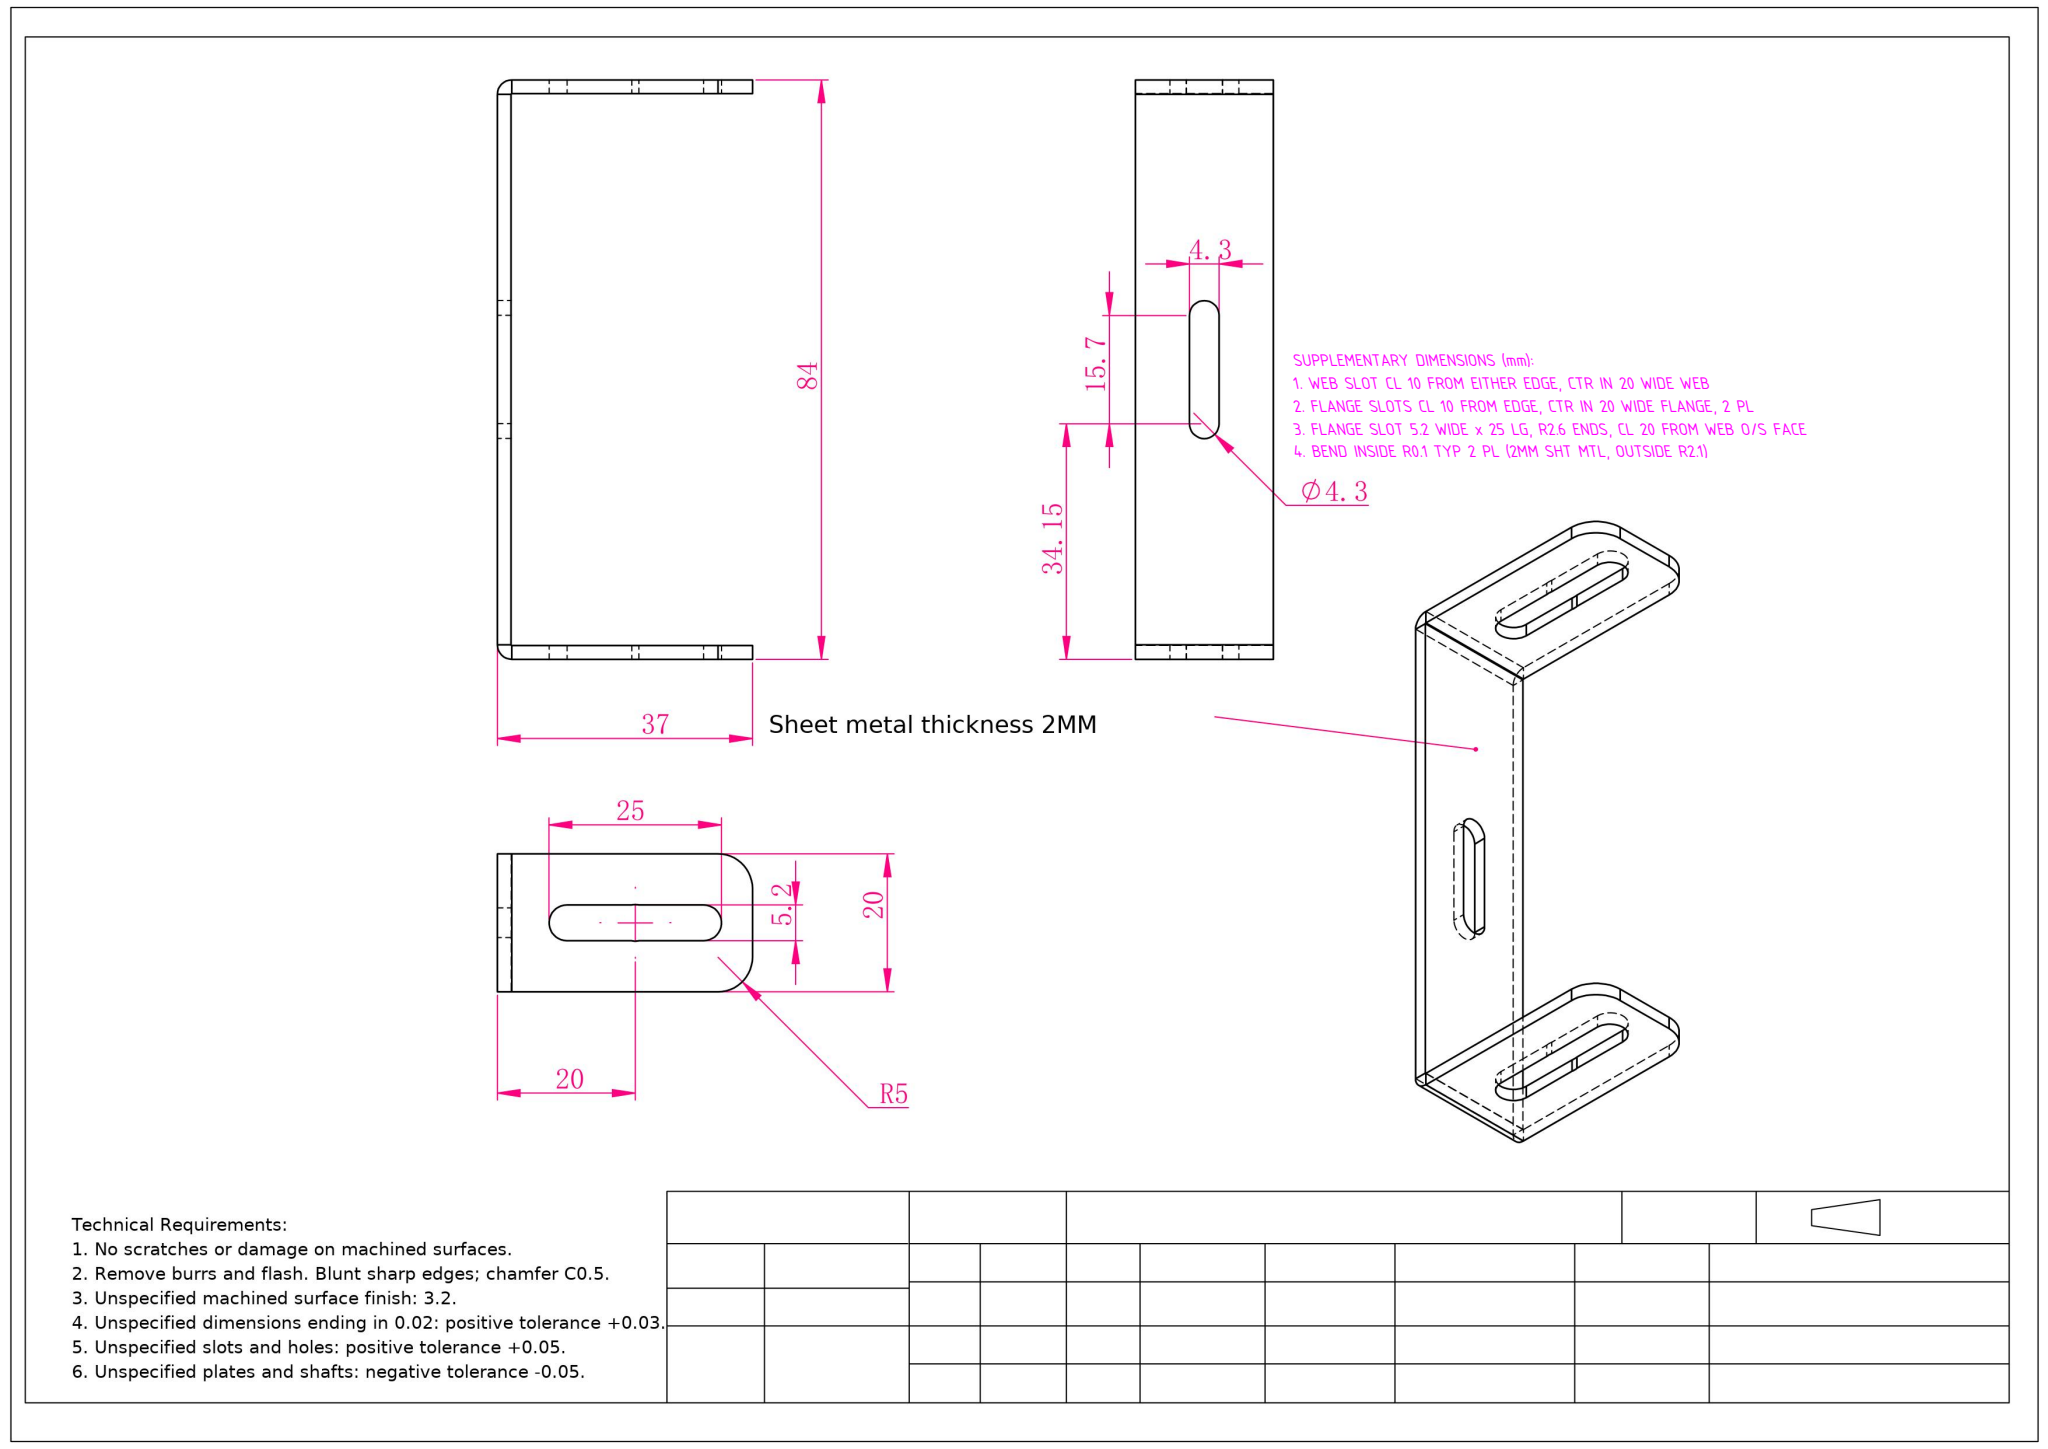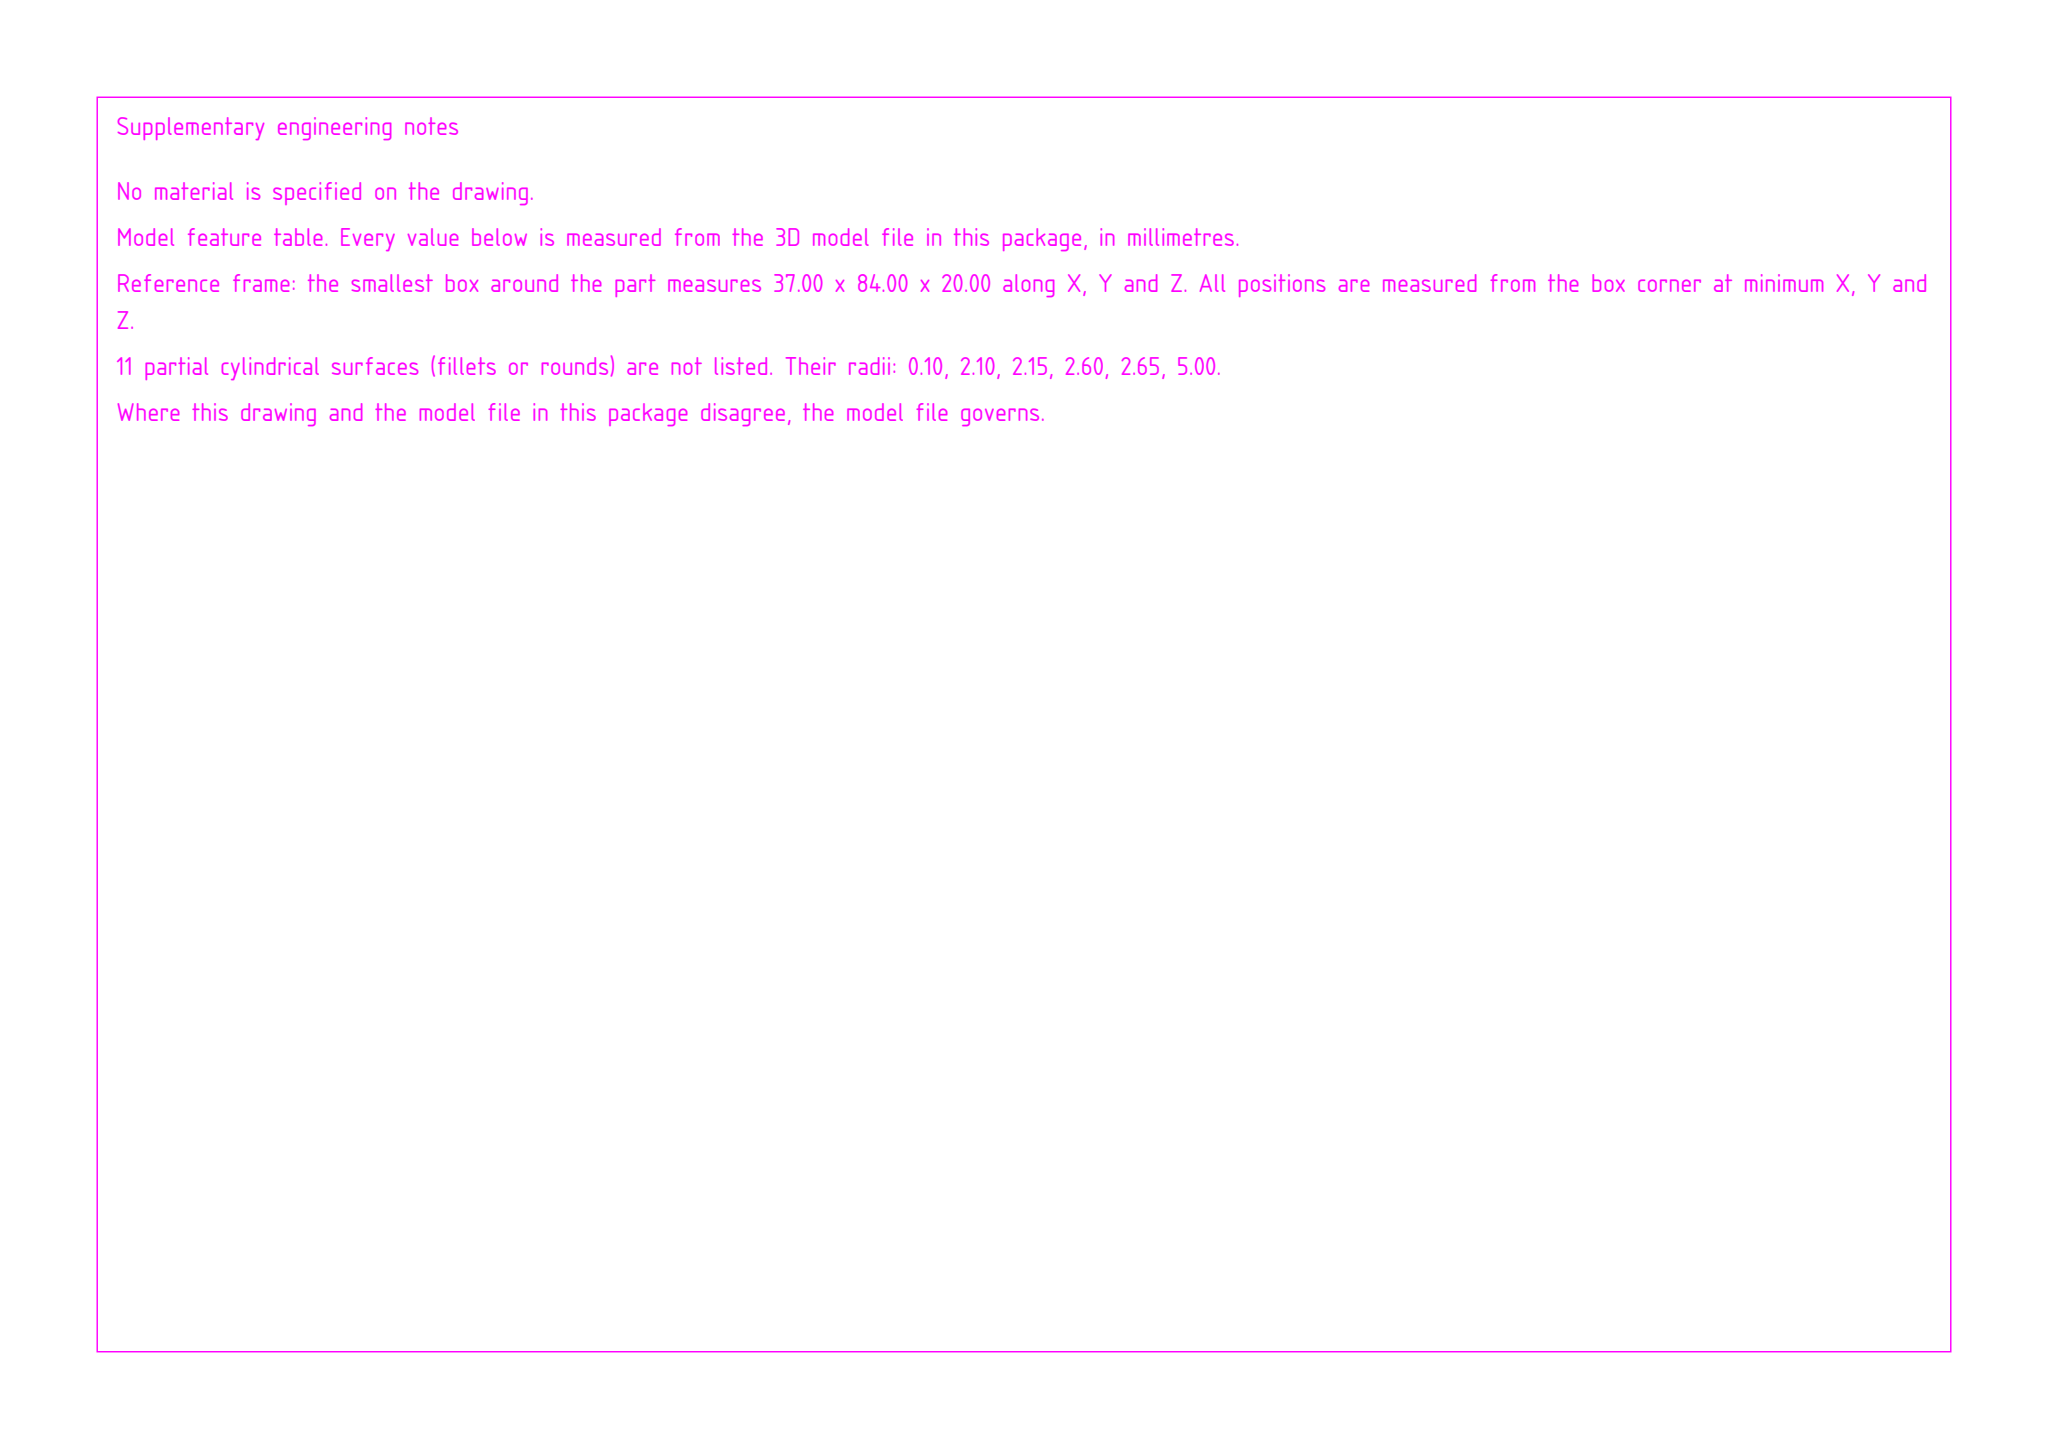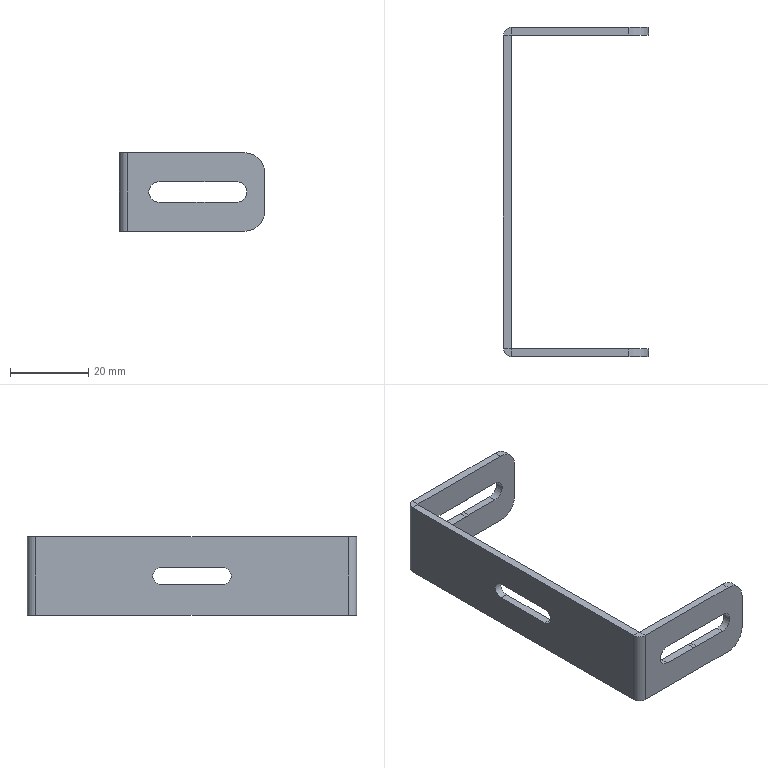Part | SolidWorks | mm | 1 solid | 48 faces | box 37 x 84 x 20 mm | volume 5418 mm3 | plane 28 | cylinder 20 | commonest cylinder face diameters 5.3 x6 10 x4 5.2 x4 0.2 x2 4.2 x2 4.3 x2